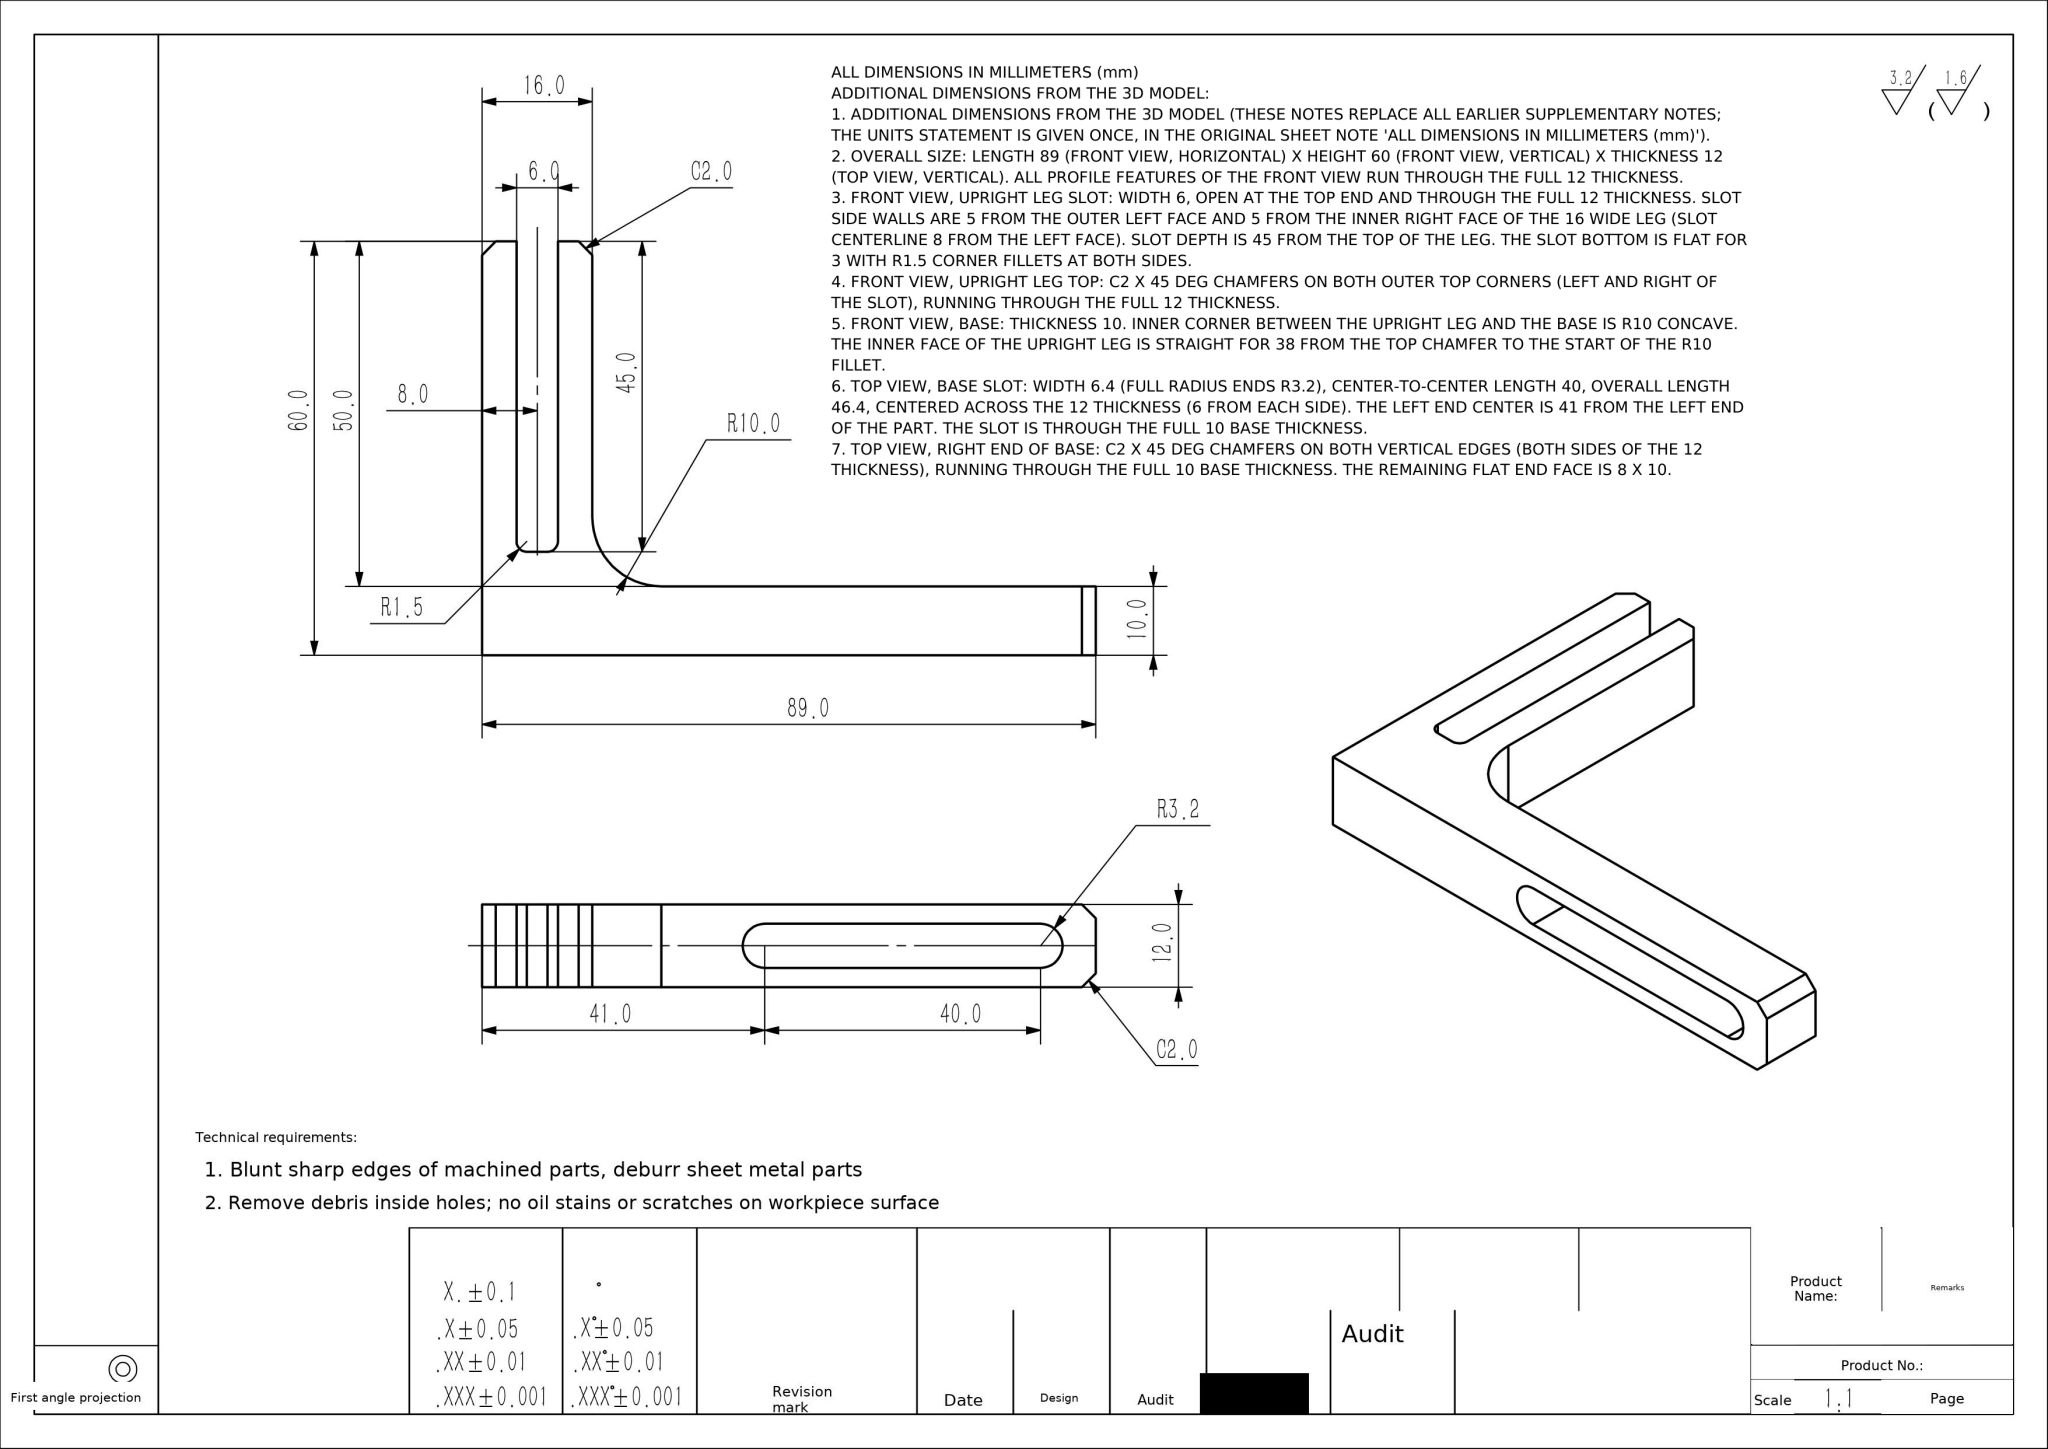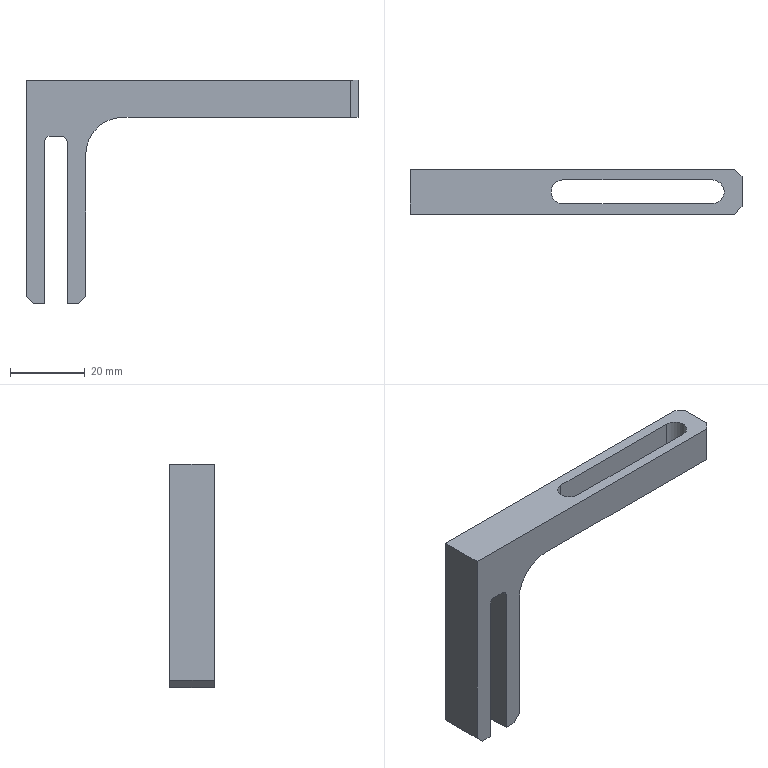Part | NX | mm | Right-Angle Slotted Post Bracket | 1 solid | 24 faces | box 89 x 12 x 60 mm | volume 14339 mm3 | plane 18 | cylinder 6 | commonest cylinder face diameters 6.4 x3 3 x2 20 x1
STEP:
#1=COLOUR_RGB('',1.,1.,1.);
#2=FILL_AREA_STYLE_COLOUR('',#1);
#3=FILL_AREA_STYLE('',(#2));
#4=SURFACE_STYLE_FILL_AREA(#3);
#5=SURFACE_SIDE_STYLE('',(#4));
#6=SURFACE_STYLE_USAGE(.BOTH.,#5);
#7=PRESENTATION_STYLE_ASSIGNMENT((#6));
#8=CARTESIAN_POINT('',(-6.7,6.,30.));
#9=VERTEX_POINT('',#8);
#10=CARTESIAN_POINT('',(-3.5,9.2,30.));
#11=VERTEX_POINT('',#10);
#12=CARTESIAN_POINT('',(-3.5,6.,30.));
#13=DIRECTION('',(-0.,0.,-1.));
#14=DIRECTION('',(-1.,0.,0.));
#15=AXIS2_PLACEMENT_3D('',#12,#13,#14);
#16=CIRCLE('',#15,3.2);
#17=EDGE_CURVE('',#9,#11,#16,.T.);
#18=ORIENTED_EDGE('',*,*,#17,.F.);
#19=CARTESIAN_POINT('',(-6.7,6.,20.));
#20=VERTEX_POINT('',#19);
#21=CARTESIAN_POINT('',(-6.7,6.,30.));
#22=DIRECTION('',(-0.,0.,-1.));
#23=VECTOR('',#22,1000.);
#24=LINE('',#21,#23);
#25=EDGE_CURVE('',#9,#20,#24,.T.);
#26=ORIENTED_EDGE('',*,*,#25,.T.);
#27=CARTESIAN_POINT('',(-3.5,9.2,20.));
#28=VERTEX_POINT('',#27);
#29=CARTESIAN_POINT('',(-3.5,6.,20.));
#30=DIRECTION('',(-0.,0.,-1.));
#31=DIRECTION('',(-1.,0.,0.));
#32=AXIS2_PLACEMENT_3D('',#29,#30,#31);
#33=CIRCLE('',#32,3.2);
#34=EDGE_CURVE('',#20,#28,#33,.T.);
#35=ORIENTED_EDGE('',*,*,#34,.T.);
#36=CARTESIAN_POINT('',(-3.5,9.2,30.));
#37=DIRECTION('',(-0.,0.,-1.));
#38=VECTOR('',#37,1000.);
#39=LINE('',#36,#38);
#40=EDGE_CURVE('',#11,#28,#39,.T.);
#41=ORIENTED_EDGE('',*,*,#40,.F.);
#42=EDGE_LOOP('',(#18,#26,#35,#41));
#43=FACE_OUTER_BOUND('',#42,.T.);
#44=CARTESIAN_POINT('',(-3.5,6.,30.));
#45=DIRECTION('',(-0.,0.,-1.));
#46=DIRECTION('',(-1.,0.,0.));
#47=AXIS2_PLACEMENT_3D('',#44,#45,#46);
#48=CYLINDRICAL_SURFACE('',#47,3.2);
#49=ADVANCED_FACE('',(#43),#48,.F.);
#50=CARTESIAN_POINT('',(-39.5,0.,-30.));
#51=VERTEX_POINT('',#50);
#52=CARTESIAN_POINT('',(-42.5,0.,-30.));
#53=VERTEX_POINT('',#52);
#54=CARTESIAN_POINT('',(-44.5,0.,-30.));
#55=DIRECTION('',(-1.,0.,0.));
#56=VECTOR('',#55,1000.);
#57=LINE('',#54,#56);
#58=EDGE_CURVE('',#51,#53,#57,.T.);
#59=ORIENTED_EDGE('',*,*,#58,.T.);
#60=CARTESIAN_POINT('',(-42.5,12.,-30.));
#61=VERTEX_POINT('',#60);
#62=CARTESIAN_POINT('',(-42.5,12.,-30.));
#63=DIRECTION('',(0.,1.,0.));
#64=VECTOR('',#63,1000.);
#65=LINE('',#62,#64);
#66=EDGE_CURVE('',#53,#61,#65,.T.);
#67=ORIENTED_EDGE('',*,*,#66,.T.);
#68=CARTESIAN_POINT('',(-39.5,12.,-30.));
#69=VERTEX_POINT('',#68);
#70=CARTESIAN_POINT('',(-44.5,12.,-30.));
#71=DIRECTION('',(-1.,0.,0.));
#72=VECTOR('',#71,1000.);
#73=LINE('',#70,#72);
#74=EDGE_CURVE('',#69,#61,#73,.T.);
#75=ORIENTED_EDGE('',*,*,#74,.F.);
#76=CARTESIAN_POINT('',(-39.5,0.,-30.));
#77=DIRECTION('',(0.,1.,0.));
#78=VECTOR('',#77,1000.);
#79=LINE('',#76,#78);
#80=EDGE_CURVE('',#51,#69,#79,.T.);
#81=ORIENTED_EDGE('',*,*,#80,.F.);
#82=EDGE_LOOP('',(#59,#67,#75,#81));
#83=FACE_OUTER_BOUND('',#82,.T.);
#84=CARTESIAN_POINT('',(-44.5,12.,-30.));
#85=DIRECTION('',(0.,0.,1.));
#86=DIRECTION('',(1.,0.,0.));
#87=AXIS2_PLACEMENT_3D('',#84,#85,#86);
#88=PLANE('',#87);
#89=ADVANCED_FACE('',(#83),#88,.F.);
#90=CARTESIAN_POINT('',(44.5,10.,30.));
#91=VERTEX_POINT('',#90);
#92=CARTESIAN_POINT('',(44.5,2.,30.));
#93=VERTEX_POINT('',#92);
#94=CARTESIAN_POINT('',(44.5,12.,30.));
#95=DIRECTION('',(0.,-1.,0.));
#96=VECTOR('',#95,1000.);
#97=LINE('',#94,#96);
#98=EDGE_CURVE('',#91,#93,#97,.T.);
#99=ORIENTED_EDGE('',*,*,#98,.T.);
#100=CARTESIAN_POINT('',(44.5,2.,20.));
#101=VERTEX_POINT('',#100);
#102=CARTESIAN_POINT('',(44.5,2.,20.));
#103=DIRECTION('',(0.,0.,-1.));
#104=VECTOR('',#103,1000.);
#105=LINE('',#102,#104);
#106=EDGE_CURVE('',#93,#101,#105,.T.);
#107=ORIENTED_EDGE('',*,*,#106,.T.);
#108=CARTESIAN_POINT('',(44.5,10.,20.));
#109=VERTEX_POINT('',#108);
#110=CARTESIAN_POINT('',(44.5,0.,20.));
#111=DIRECTION('',(0.,1.,0.));
#112=VECTOR('',#111,1000.);
#113=LINE('',#110,#112);
#114=EDGE_CURVE('',#101,#109,#113,.T.);
#115=ORIENTED_EDGE('',*,*,#114,.T.);
#116=CARTESIAN_POINT('',(44.5,10.,30.));
#117=DIRECTION('',(0.,0.,1.));
#118=VECTOR('',#117,1000.);
#119=LINE('',#116,#118);
#120=EDGE_CURVE('',#109,#91,#119,.T.);
#121=ORIENTED_EDGE('',*,*,#120,.T.);
#122=EDGE_LOOP('',(#99,#107,#115,#121));
#123=FACE_OUTER_BOUND('',#122,.T.);
#124=CARTESIAN_POINT('',(44.5,12.,30.));
#125=DIRECTION('',(-1.,0.,0.));
#126=DIRECTION('',(0.,0.,1.));
#127=AXIS2_PLACEMENT_3D('',#124,#125,#126);
#128=PLANE('',#127);
#129=ADVANCED_FACE('',(#123),#128,.F.);
#130=CARTESIAN_POINT('',(-30.5,12.,-30.));
#131=VERTEX_POINT('',#130);
#132=CARTESIAN_POINT('',(-33.5,12.,-30.));
#133=VERTEX_POINT('',#132);
#134=CARTESIAN_POINT('',(-44.5,12.,-30.));
#135=DIRECTION('',(-1.,0.,0.));
#136=VECTOR('',#135,1000.);
#137=LINE('',#134,#136);
#138=EDGE_CURVE('',#131,#133,#137,.T.);
#139=ORIENTED_EDGE('',*,*,#138,.F.);
#140=CARTESIAN_POINT('',(-30.5,0.,-30.));
#141=VERTEX_POINT('',#140);
#142=CARTESIAN_POINT('',(-30.5,12.,-30.));
#143=DIRECTION('',(0.,-1.,0.));
#144=VECTOR('',#143,1000.);
#145=LINE('',#142,#144);
#146=EDGE_CURVE('',#131,#141,#145,.T.);
#147=ORIENTED_EDGE('',*,*,#146,.T.);
#148=CARTESIAN_POINT('',(-33.5,0.,-30.));
#149=VERTEX_POINT('',#148);
#150=CARTESIAN_POINT('',(-44.5,0.,-30.));
#151=DIRECTION('',(-1.,0.,0.));
#152=VECTOR('',#151,1000.);
#153=LINE('',#150,#152);
#154=EDGE_CURVE('',#141,#149,#153,.T.);
#155=ORIENTED_EDGE('',*,*,#154,.T.);
#156=CARTESIAN_POINT('',(-33.5,0.,-30.));
#157=DIRECTION('',(0.,1.,0.));
#158=VECTOR('',#157,1000.);
#159=LINE('',#156,#158);
#160=EDGE_CURVE('',#149,#133,#159,.T.);
#161=ORIENTED_EDGE('',*,*,#160,.T.);
#162=EDGE_LOOP('',(#139,#147,#155,#161));
#163=FACE_OUTER_BOUND('',#162,.T.);
#164=CARTESIAN_POINT('',(-44.5,12.,-30.));
#165=DIRECTION('',(0.,0.,1.));
#166=DIRECTION('',(1.,0.,0.));
#167=AXIS2_PLACEMENT_3D('',#164,#165,#166);
#168=PLANE('',#167);
#169=ADVANCED_FACE('',(#163),#168,.F.);
#170=CARTESIAN_POINT('',(-44.5,12.,-28.));
#171=VERTEX_POINT('',#170);
#172=CARTESIAN_POINT('',(-44.5,12.,30.));
#173=VERTEX_POINT('',#172);
#174=CARTESIAN_POINT('',(-44.5,12.,30.));
#175=DIRECTION('',(0.,0.,1.));
#176=VECTOR('',#175,1000.);
#177=LINE('',#174,#176);
#178=EDGE_CURVE('',#171,#173,#177,.T.);
#179=ORIENTED_EDGE('',*,*,#178,.F.);
#180=CARTESIAN_POINT('',(-44.5,0.,-28.));
#181=VERTEX_POINT('',#180);
#182=CARTESIAN_POINT('',(-44.5,12.,-28.));
#183=DIRECTION('',(0.,-1.,0.));
#184=VECTOR('',#183,1000.);
#185=LINE('',#182,#184);
#186=EDGE_CURVE('',#171,#181,#185,.T.);
#187=ORIENTED_EDGE('',*,*,#186,.T.);
#188=CARTESIAN_POINT('',(-44.5,0.,30.));
#189=VERTEX_POINT('',#188);
#190=CARTESIAN_POINT('',(-44.5,0.,30.));
#191=DIRECTION('',(0.,0.,1.));
#192=VECTOR('',#191,1000.);
#193=LINE('',#190,#192);
#194=EDGE_CURVE('',#181,#189,#193,.T.);
#195=ORIENTED_EDGE('',*,*,#194,.T.);
#196=CARTESIAN_POINT('',(-44.5,12.,30.));
#197=DIRECTION('',(0.,-1.,0.));
#198=VECTOR('',#197,1000.);
#199=LINE('',#196,#198);
#200=EDGE_CURVE('',#173,#189,#199,.T.);
#201=ORIENTED_EDGE('',*,*,#200,.F.);
#202=EDGE_LOOP('',(#179,#187,#195,#201));
#203=FACE_OUTER_BOUND('',#202,.T.);
#204=CARTESIAN_POINT('',(-44.5,12.,30.));
#205=DIRECTION('',(1.,0.,0.));
#206=DIRECTION('',(0.,0.,-1.));
#207=AXIS2_PLACEMENT_3D('',#204,#205,#206);
#208=PLANE('',#207);
#209=ADVANCED_FACE('',(#203),#208,.F.);
#210=CARTESIAN_POINT('',(36.5,9.2,30.));
#211=VERTEX_POINT('',#210);
#212=CARTESIAN_POINT('',(36.5,9.2,30.));
#213=DIRECTION('',(1.,0.,0.));
#214=VECTOR('',#213,1000.);
#215=LINE('',#212,#214);
#216=EDGE_CURVE('',#11,#211,#215,.T.);
#217=ORIENTED_EDGE('',*,*,#216,.T.);
#218=CARTESIAN_POINT('',(36.5,2.8,30.));
#219=VERTEX_POINT('',#218);
#220=CARTESIAN_POINT('',(36.5,6.,30.));
#221=DIRECTION('',(-0.,0.,-1.));
#222=DIRECTION('',(-1.,0.,0.));
#223=AXIS2_PLACEMENT_3D('',#220,#221,#222);
#224=CIRCLE('',#223,3.2);
#225=EDGE_CURVE('',#211,#219,#224,.T.);
#226=ORIENTED_EDGE('',*,*,#225,.T.);
#227=CARTESIAN_POINT('',(-3.5,2.8,30.));
#228=VERTEX_POINT('',#227);
#229=CARTESIAN_POINT('',(36.5,2.8,30.));
#230=DIRECTION('',(-1.,0.,0.));
#231=VECTOR('',#230,1000.);
#232=LINE('',#229,#231);
#233=EDGE_CURVE('',#219,#228,#232,.T.);
#234=ORIENTED_EDGE('',*,*,#233,.T.);
#235=CARTESIAN_POINT('',(-3.5,6.,30.));
#236=DIRECTION('',(-0.,0.,-1.));
#237=DIRECTION('',(-1.,0.,0.));
#238=AXIS2_PLACEMENT_3D('',#235,#236,#237);
#239=CIRCLE('',#238,3.2);
#240=EDGE_CURVE('',#228,#9,#239,.T.);
#241=ORIENTED_EDGE('',*,*,#240,.T.);
#242=ORIENTED_EDGE('',*,*,#17,.T.);
#243=EDGE_LOOP('',(#217,#226,#234,#241,#242));
#244=FACE_BOUND('',#243,.T.);
#245=CARTESIAN_POINT('',(42.5,0.,30.));
#246=VERTEX_POINT('',#245);
#247=CARTESIAN_POINT('',(-44.5,0.,30.));
#248=DIRECTION('',(1.,0.,0.));
#249=VECTOR('',#248,1000.);
#250=LINE('',#247,#249);
#251=EDGE_CURVE('',#189,#246,#250,.T.);
#252=ORIENTED_EDGE('',*,*,#251,.T.);
#253=CARTESIAN_POINT('',(44.5,2.,30.));
#254=DIRECTION('',(0.7071,0.7071,0.));
#255=VECTOR('',#254,1000.);
#256=LINE('',#253,#255);
#257=EDGE_CURVE('',#246,#93,#256,.T.);
#258=ORIENTED_EDGE('',*,*,#257,.T.);
#259=ORIENTED_EDGE('',*,*,#98,.F.);
#260=CARTESIAN_POINT('',(42.5,12.,30.));
#261=VERTEX_POINT('',#260);
#262=CARTESIAN_POINT('',(42.5,12.,30.));
#263=DIRECTION('',(-0.7071,0.7071,0.));
#264=VECTOR('',#263,1000.);
#265=LINE('',#262,#264);
#266=EDGE_CURVE('',#91,#261,#265,.T.);
#267=ORIENTED_EDGE('',*,*,#266,.T.);
#268=CARTESIAN_POINT('',(-44.5,12.,30.));
#269=DIRECTION('',(1.,0.,0.));
#270=VECTOR('',#269,1000.);
#271=LINE('',#268,#270);
#272=EDGE_CURVE('',#173,#261,#271,.T.);
#273=ORIENTED_EDGE('',*,*,#272,.F.);
#274=ORIENTED_EDGE('',*,*,#200,.T.);
#275=EDGE_LOOP('',(#252,#258,#259,#267,#273,#274));
#276=FACE_OUTER_BOUND('',#275,.T.);
#277=CARTESIAN_POINT('',(-44.5,12.,30.));
#278=DIRECTION('',(0.,0.,-1.));
#279=DIRECTION('',(-1.,0.,0.));
#280=AXIS2_PLACEMENT_3D('',#277,#278,#279);
#281=PLANE('',#280);
#282=ADVANCED_FACE('',(#244,#276),#281,.F.);
#283=ORIENTED_EDGE('',*,*,#74,.T.);
#284=CARTESIAN_POINT('',(-44.5,12.,-28.));
#285=DIRECTION('',(-0.7071,0.,0.7071));
#286=VECTOR('',#285,1000.);
#287=LINE('',#284,#286);
#288=EDGE_CURVE('',#61,#171,#287,.T.);
#289=ORIENTED_EDGE('',*,*,#288,.T.);
#290=ORIENTED_EDGE('',*,*,#178,.T.);
#291=ORIENTED_EDGE('',*,*,#272,.T.);
#292=CARTESIAN_POINT('',(42.5,12.,20.));
#293=VERTEX_POINT('',#292);
#294=CARTESIAN_POINT('',(42.5,12.,0.));
#295=DIRECTION('',(0.,0.,-1.));
#296=VECTOR('',#295,1000.);
#297=LINE('',#294,#296);
#298=EDGE_CURVE('',#261,#293,#297,.T.);
#299=ORIENTED_EDGE('',*,*,#298,.T.);
#300=CARTESIAN_POINT('',(-18.5,12.,20.));
#301=VERTEX_POINT('',#300);
#302=CARTESIAN_POINT('',(44.5,12.,20.));
#303=DIRECTION('',(1.,0.,-0.));
#304=VECTOR('',#303,1000.);
#305=LINE('',#302,#304);
#306=EDGE_CURVE('',#301,#293,#305,.T.);
#307=ORIENTED_EDGE('',*,*,#306,.F.);
#308=CARTESIAN_POINT('',(-28.5,12.,10.));
#309=VERTEX_POINT('',#308);
#310=CARTESIAN_POINT('',(-18.5,12.,10.));
#311=DIRECTION('',(0.,-1.,0.));
#312=DIRECTION('',(0.,0.,-1.));
#313=AXIS2_PLACEMENT_3D('',#310,#311,#312);
#314=CIRCLE('',#313,10.);
#315=EDGE_CURVE('',#301,#309,#314,.T.);
#316=ORIENTED_EDGE('',*,*,#315,.T.);
#317=CARTESIAN_POINT('',(-28.5,12.,-28.));
#318=VERTEX_POINT('',#317);
#319=CARTESIAN_POINT('',(-28.5,12.,-30.));
#320=DIRECTION('',(0.,0.,1.));
#321=VECTOR('',#320,1000.);
#322=LINE('',#319,#321);
#323=EDGE_CURVE('',#318,#309,#322,.T.);
#324=ORIENTED_EDGE('',*,*,#323,.F.);
#325=CARTESIAN_POINT('',(-28.5,12.,-28.));
#326=DIRECTION('',(-0.7071,0.,-0.7071));
#327=VECTOR('',#326,1000.);
#328=LINE('',#325,#327);
#329=EDGE_CURVE('',#318,#131,#328,.T.);
#330=ORIENTED_EDGE('',*,*,#329,.T.);
#331=ORIENTED_EDGE('',*,*,#138,.T.);
#332=CARTESIAN_POINT('',(-33.5,12.,13.5));
#333=VERTEX_POINT('',#332);
#334=CARTESIAN_POINT('',(-33.5,12.,-30.));
#335=DIRECTION('',(0.,0.,-1.));
#336=VECTOR('',#335,1000.);
#337=LINE('',#334,#336);
#338=EDGE_CURVE('',#333,#133,#337,.T.);
#339=ORIENTED_EDGE('',*,*,#338,.F.);
#340=CARTESIAN_POINT('',(-35.,12.,15.));
#341=VERTEX_POINT('',#340);
#342=CARTESIAN_POINT('',(-35.,12.,13.5));
#343=DIRECTION('',(0.,-1.,0.));
#344=DIRECTION('',(0.,0.,-1.));
#345=AXIS2_PLACEMENT_3D('',#342,#343,#344);
#346=CIRCLE('',#345,1.5);
#347=EDGE_CURVE('',#333,#341,#346,.T.);
#348=ORIENTED_EDGE('',*,*,#347,.T.);
#349=CARTESIAN_POINT('',(-38.,12.,15.));
#350=VERTEX_POINT('',#349);
#351=CARTESIAN_POINT('',(-39.5,12.,15.));
#352=DIRECTION('',(1.,0.,0.));
#353=VECTOR('',#352,1000.);
#354=LINE('',#351,#353);
#355=EDGE_CURVE('',#350,#341,#354,.T.);
#356=ORIENTED_EDGE('',*,*,#355,.F.);
#357=CARTESIAN_POINT('',(-39.5,12.,13.5));
#358=VERTEX_POINT('',#357);
#359=CARTESIAN_POINT('',(-38.,12.,13.5));
#360=DIRECTION('',(0.,-1.,0.));
#361=DIRECTION('',(0.,0.,-1.));
#362=AXIS2_PLACEMENT_3D('',#359,#360,#361);
#363=CIRCLE('',#362,1.5);
#364=EDGE_CURVE('',#350,#358,#363,.T.);
#365=ORIENTED_EDGE('',*,*,#364,.T.);
#366=CARTESIAN_POINT('',(-39.5,12.,-30.));
#367=DIRECTION('',(0.,0.,1.));
#368=VECTOR('',#367,1000.);
#369=LINE('',#366,#368);
#370=EDGE_CURVE('',#69,#358,#369,.T.);
#371=ORIENTED_EDGE('',*,*,#370,.F.);
#372=EDGE_LOOP('',(#283,#289,#290,#291,#299,#307,#316,#324,#330,#331,#339,#348,#356,#365,#371));
#373=FACE_OUTER_BOUND('',#372,.T.);
#374=CARTESIAN_POINT('',(0.,12.,0.));
#375=DIRECTION('',(0.,-1.,0.));
#376=DIRECTION('',(0.,0.,-1.));
#377=AXIS2_PLACEMENT_3D('',#374,#375,#376);
#378=PLANE('',#377);
#379=ADVANCED_FACE('',(#373),#378,.F.);
#380=ORIENTED_EDGE('',*,*,#194,.F.);
#381=CARTESIAN_POINT('',(-36.25,0.,-36.25));
#382=DIRECTION('',(0.7071,0.,-0.7071));
#383=VECTOR('',#382,1000.);
#384=LINE('',#381,#383);
#385=EDGE_CURVE('',#181,#53,#384,.T.);
#386=ORIENTED_EDGE('',*,*,#385,.T.);
#387=ORIENTED_EDGE('',*,*,#58,.F.);
#388=CARTESIAN_POINT('',(-39.5,0.,13.5));
#389=VERTEX_POINT('',#388);
#390=CARTESIAN_POINT('',(-39.5,0.,-30.));
#391=DIRECTION('',(0.,0.,1.));
#392=VECTOR('',#391,1000.);
#393=LINE('',#390,#392);
#394=EDGE_CURVE('',#51,#389,#393,.T.);
#395=ORIENTED_EDGE('',*,*,#394,.T.);
#396=CARTESIAN_POINT('',(-38.,0.,15.));
#397=VERTEX_POINT('',#396);
#398=CARTESIAN_POINT('',(-38.,0.,13.5));
#399=DIRECTION('',(0.,1.,0.));
#400=DIRECTION('',(0.,0.,-1.));
#401=AXIS2_PLACEMENT_3D('',#398,#399,#400);
#402=CIRCLE('',#401,1.5);
#403=EDGE_CURVE('',#389,#397,#402,.T.);
#404=ORIENTED_EDGE('',*,*,#403,.T.);
#405=CARTESIAN_POINT('',(-35.,0.,15.));
#406=VERTEX_POINT('',#405);
#407=CARTESIAN_POINT('',(-39.5,0.,15.));
#408=DIRECTION('',(1.,0.,0.));
#409=VECTOR('',#408,1000.);
#410=LINE('',#407,#409);
#411=EDGE_CURVE('',#397,#406,#410,.T.);
#412=ORIENTED_EDGE('',*,*,#411,.T.);
#413=CARTESIAN_POINT('',(-33.5,0.,13.5));
#414=VERTEX_POINT('',#413);
#415=CARTESIAN_POINT('',(-35.,0.,13.5));
#416=DIRECTION('',(0.,1.,0.));
#417=DIRECTION('',(0.,0.,-1.));
#418=AXIS2_PLACEMENT_3D('',#415,#416,#417);
#419=CIRCLE('',#418,1.5);
#420=EDGE_CURVE('',#406,#414,#419,.T.);
#421=ORIENTED_EDGE('',*,*,#420,.T.);
#422=CARTESIAN_POINT('',(-33.5,0.,-30.));
#423=DIRECTION('',(0.,0.,-1.));
#424=VECTOR('',#423,1000.);
#425=LINE('',#422,#424);
#426=EDGE_CURVE('',#414,#149,#425,.T.);
#427=ORIENTED_EDGE('',*,*,#426,.T.);
#428=ORIENTED_EDGE('',*,*,#154,.F.);
#429=CARTESIAN_POINT('',(-28.5,0.,-28.));
#430=VERTEX_POINT('',#429);
#431=CARTESIAN_POINT('',(-0.25,0.,0.25));
#432=DIRECTION('',(0.7071,0.,0.7071));
#433=VECTOR('',#432,1000.);
#434=LINE('',#431,#433);
#435=EDGE_CURVE('',#141,#430,#434,.T.);
#436=ORIENTED_EDGE('',*,*,#435,.T.);
#437=CARTESIAN_POINT('',(-28.5,0.,10.));
#438=VERTEX_POINT('',#437);
#439=CARTESIAN_POINT('',(-28.5,0.,-30.));
#440=DIRECTION('',(0.,0.,1.));
#441=VECTOR('',#440,1000.);
#442=LINE('',#439,#441);
#443=EDGE_CURVE('',#430,#438,#442,.T.);
#444=ORIENTED_EDGE('',*,*,#443,.T.);
#445=CARTESIAN_POINT('',(-18.5,0.,20.));
#446=VERTEX_POINT('',#445);
#447=CARTESIAN_POINT('',(-18.5,0.,10.));
#448=DIRECTION('',(0.,1.,0.));
#449=DIRECTION('',(0.,0.,-1.));
#450=AXIS2_PLACEMENT_3D('',#447,#448,#449);
#451=CIRCLE('',#450,10.);
#452=EDGE_CURVE('',#438,#446,#451,.T.);
#453=ORIENTED_EDGE('',*,*,#452,.T.);
#454=CARTESIAN_POINT('',(42.5,0.,20.));
#455=VERTEX_POINT('',#454);
#456=CARTESIAN_POINT('',(44.5,0.,20.));
#457=DIRECTION('',(1.,0.,-0.));
#458=VECTOR('',#457,1000.);
#459=LINE('',#456,#458);
#460=EDGE_CURVE('',#446,#455,#459,.T.);
#461=ORIENTED_EDGE('',*,*,#460,.T.);
#462=CARTESIAN_POINT('',(42.5,0.,30.));
#463=DIRECTION('',(0.,0.,1.));
#464=VECTOR('',#463,1000.);
#465=LINE('',#462,#464);
#466=EDGE_CURVE('',#455,#246,#465,.T.);
#467=ORIENTED_EDGE('',*,*,#466,.T.);
#468=ORIENTED_EDGE('',*,*,#251,.F.);
#469=EDGE_LOOP('',(#380,#386,#387,#395,#404,#412,#421,#427,#428,#436,#444,#453,#461,#467,#468));
#470=FACE_OUTER_BOUND('',#469,.T.);
#471=CARTESIAN_POINT('',(0.,0.,0.));
#472=DIRECTION('',(0.,-1.,0.));
#473=DIRECTION('',(0.,0.,-1.));
#474=AXIS2_PLACEMENT_3D('',#471,#472,#473);
#475=PLANE('',#474);
#476=ADVANCED_FACE('',(#470),#475,.T.);
#477=CARTESIAN_POINT('',(36.5,2.8,20.));
#478=VERTEX_POINT('',#477);
#479=CARTESIAN_POINT('',(-3.5,2.8,20.));
#480=VERTEX_POINT('',#479);
#481=CARTESIAN_POINT('',(36.5,2.8,20.));
#482=DIRECTION('',(-1.,0.,0.));
#483=VECTOR('',#482,1000.);
#484=LINE('',#481,#483);
#485=EDGE_CURVE('',#478,#480,#484,.T.);
#486=ORIENTED_EDGE('',*,*,#485,.F.);
#487=CARTESIAN_POINT('',(36.5,9.2,20.));
#488=VERTEX_POINT('',#487);
#489=CARTESIAN_POINT('',(36.5,6.,20.));
#490=DIRECTION('',(-0.,0.,-1.));
#491=DIRECTION('',(-1.,0.,0.));
#492=AXIS2_PLACEMENT_3D('',#489,#490,#491);
#493=CIRCLE('',#492,3.2);
#494=EDGE_CURVE('',#488,#478,#493,.T.);
#495=ORIENTED_EDGE('',*,*,#494,.F.);
#496=CARTESIAN_POINT('',(36.5,9.2,20.));
#497=DIRECTION('',(1.,0.,0.));
#498=VECTOR('',#497,1000.);
#499=LINE('',#496,#498);
#500=EDGE_CURVE('',#28,#488,#499,.T.);
#501=ORIENTED_EDGE('',*,*,#500,.F.);
#502=ORIENTED_EDGE('',*,*,#34,.F.);
#503=CARTESIAN_POINT('',(-3.5,6.,20.));
#504=DIRECTION('',(-0.,0.,-1.));
#505=DIRECTION('',(-1.,0.,0.));
#506=AXIS2_PLACEMENT_3D('',#503,#504,#505);
#507=CIRCLE('',#506,3.2);
#508=EDGE_CURVE('',#480,#20,#507,.T.);
#509=ORIENTED_EDGE('',*,*,#508,.F.);
#510=EDGE_LOOP('',(#486,#495,#501,#502,#509));
#511=FACE_BOUND('',#510,.T.);
#512=ORIENTED_EDGE('',*,*,#114,.F.);
#513=CARTESIAN_POINT('',(44.5,2.,20.));
#514=DIRECTION('',(-0.7071,-0.7071,0.));
#515=VECTOR('',#514,1000.);
#516=LINE('',#513,#515);
#517=EDGE_CURVE('',#101,#455,#516,.T.);
#518=ORIENTED_EDGE('',*,*,#517,.T.);
#519=ORIENTED_EDGE('',*,*,#460,.F.);
#520=CARTESIAN_POINT('',(-18.5,12.,20.));
#521=DIRECTION('',(0.,1.,0.));
#522=VECTOR('',#521,1000.);
#523=LINE('',#520,#522);
#524=EDGE_CURVE('',#446,#301,#523,.T.);
#525=ORIENTED_EDGE('',*,*,#524,.T.);
#526=ORIENTED_EDGE('',*,*,#306,.T.);
#527=CARTESIAN_POINT('',(42.5,12.,20.));
#528=DIRECTION('',(0.7071,-0.7071,-0.));
#529=VECTOR('',#528,1000.);
#530=LINE('',#527,#529);
#531=EDGE_CURVE('',#293,#109,#530,.T.);
#532=ORIENTED_EDGE('',*,*,#531,.T.);
#533=EDGE_LOOP('',(#512,#518,#519,#525,#526,#532));
#534=FACE_OUTER_BOUND('',#533,.T.);
#535=CARTESIAN_POINT('',(44.5,0.,20.));
#536=DIRECTION('',(0.,0.,1.));
#537=DIRECTION('',(1.,0.,-0.));
#538=AXIS2_PLACEMENT_3D('',#535,#536,#537);
#539=PLANE('',#538);
#540=ADVANCED_FACE('',(#511,#534),#539,.F.);
#541=ORIENTED_EDGE('',*,*,#443,.F.);
#542=CARTESIAN_POINT('',(-28.5,0.,-28.));
#543=DIRECTION('',(0.,1.,0.));
#544=VECTOR('',#543,1000.);
#545=LINE('',#542,#544);
#546=EDGE_CURVE('',#430,#318,#545,.T.);
#547=ORIENTED_EDGE('',*,*,#546,.T.);
#548=ORIENTED_EDGE('',*,*,#323,.T.);
#549=CARTESIAN_POINT('',(-28.5,0.,10.));
#550=DIRECTION('',(0.,-1.,0.));
#551=VECTOR('',#550,1000.);
#552=LINE('',#549,#551);
#553=EDGE_CURVE('',#309,#438,#552,.T.);
#554=ORIENTED_EDGE('',*,*,#553,.T.);
#555=EDGE_LOOP('',(#541,#547,#548,#554));
#556=FACE_OUTER_BOUND('',#555,.T.);
#557=CARTESIAN_POINT('',(-28.5,0.,-30.));
#558=DIRECTION('',(-1.,0.,0.));
#559=DIRECTION('',(0.,0.,1.));
#560=AXIS2_PLACEMENT_3D('',#557,#558,#559);
#561=PLANE('',#560);
#562=ADVANCED_FACE('',(#556),#561,.F.);
#563=ORIENTED_EDGE('',*,*,#452,.F.);
#564=ORIENTED_EDGE('',*,*,#553,.F.);
#565=ORIENTED_EDGE('',*,*,#315,.F.);
#566=ORIENTED_EDGE('',*,*,#524,.F.);
#567=EDGE_LOOP('',(#563,#564,#565,#566));
#568=FACE_OUTER_BOUND('',#567,.T.);
#569=CARTESIAN_POINT('',(-18.5,0.,10.));
#570=DIRECTION('',(0.,-1.,0.));
#571=DIRECTION('',(0.,0.,-1.));
#572=AXIS2_PLACEMENT_3D('',#569,#570,#571);
#573=CYLINDRICAL_SURFACE('',#572,10.);
#574=ADVANCED_FACE('',(#568),#573,.F.);
#575=ORIENTED_EDGE('',*,*,#370,.T.);
#576=CARTESIAN_POINT('',(-39.5,0.,13.5));
#577=DIRECTION('',(0.,-1.,0.));
#578=VECTOR('',#577,1000.);
#579=LINE('',#576,#578);
#580=EDGE_CURVE('',#358,#389,#579,.T.);
#581=ORIENTED_EDGE('',*,*,#580,.T.);
#582=ORIENTED_EDGE('',*,*,#394,.F.);
#583=ORIENTED_EDGE('',*,*,#80,.T.);
#584=EDGE_LOOP('',(#575,#581,#582,#583));
#585=FACE_OUTER_BOUND('',#584,.T.);
#586=CARTESIAN_POINT('',(-39.5,0.,-30.));
#587=DIRECTION('',(-1.,0.,0.));
#588=DIRECTION('',(0.,0.,1.));
#589=AXIS2_PLACEMENT_3D('',#586,#587,#588);
#590=PLANE('',#589);
#591=ADVANCED_FACE('',(#585),#590,.F.);
#592=ORIENTED_EDGE('',*,*,#426,.F.);
#593=CARTESIAN_POINT('',(-33.5,12.,13.5));
#594=DIRECTION('',(0.,1.,0.));
#595=VECTOR('',#594,1000.);
#596=LINE('',#593,#595);
#597=EDGE_CURVE('',#414,#333,#596,.T.);
#598=ORIENTED_EDGE('',*,*,#597,.T.);
#599=ORIENTED_EDGE('',*,*,#338,.T.);
#600=ORIENTED_EDGE('',*,*,#160,.F.);
#601=EDGE_LOOP('',(#592,#598,#599,#600));
#602=FACE_OUTER_BOUND('',#601,.T.);
#603=CARTESIAN_POINT('',(-33.5,0.,-30.));
#604=DIRECTION('',(1.,0.,0.));
#605=DIRECTION('',(0.,0.,-1.));
#606=AXIS2_PLACEMENT_3D('',#603,#604,#605);
#607=PLANE('',#606);
#608=ADVANCED_FACE('',(#602),#607,.F.);
#609=ORIENTED_EDGE('',*,*,#411,.F.);
#610=CARTESIAN_POINT('',(-38.,12.,15.));
#611=DIRECTION('',(0.,1.,0.));
#612=VECTOR('',#611,1000.);
#613=LINE('',#610,#612);
#614=EDGE_CURVE('',#397,#350,#613,.T.);
#615=ORIENTED_EDGE('',*,*,#614,.T.);
#616=ORIENTED_EDGE('',*,*,#355,.T.);
#617=CARTESIAN_POINT('',(-35.,0.,15.));
#618=DIRECTION('',(0.,-1.,0.));
#619=VECTOR('',#618,1000.);
#620=LINE('',#617,#619);
#621=EDGE_CURVE('',#341,#406,#620,.T.);
#622=ORIENTED_EDGE('',*,*,#621,.T.);
#623=EDGE_LOOP('',(#609,#615,#616,#622));
#624=FACE_OUTER_BOUND('',#623,.T.);
#625=CARTESIAN_POINT('',(-39.5,0.,15.));
#626=DIRECTION('',(0.,0.,1.));
#627=DIRECTION('',(1.,0.,0.));
#628=AXIS2_PLACEMENT_3D('',#625,#626,#627);
#629=PLANE('',#628);
#630=ADVANCED_FACE('',(#624),#629,.F.);
#631=ORIENTED_EDGE('',*,*,#494,.T.);
#632=CARTESIAN_POINT('',(36.5,2.8,30.));
#633=DIRECTION('',(-0.,0.,-1.));
#634=VECTOR('',#633,1000.);
#635=LINE('',#632,#634);
#636=EDGE_CURVE('',#219,#478,#635,.T.);
#637=ORIENTED_EDGE('',*,*,#636,.F.);
#638=ORIENTED_EDGE('',*,*,#225,.F.);
#639=CARTESIAN_POINT('',(36.5,9.2,30.));
#640=DIRECTION('',(-0.,0.,-1.));
#641=VECTOR('',#640,1000.);
#642=LINE('',#639,#641);
#643=EDGE_CURVE('',#211,#488,#642,.T.);
#644=ORIENTED_EDGE('',*,*,#643,.T.);
#645=EDGE_LOOP('',(#631,#637,#638,#644));
#646=FACE_OUTER_BOUND('',#645,.T.);
#647=CARTESIAN_POINT('',(36.5,6.,30.));
#648=DIRECTION('',(-0.,0.,-1.));
#649=DIRECTION('',(-1.,0.,0.));
#650=AXIS2_PLACEMENT_3D('',#647,#648,#649);
#651=CYLINDRICAL_SURFACE('',#650,3.2);
#652=ADVANCED_FACE('',(#646),#651,.F.);
#653=ORIENTED_EDGE('',*,*,#500,.T.);
#654=ORIENTED_EDGE('',*,*,#643,.F.);
#655=ORIENTED_EDGE('',*,*,#216,.F.);
#656=ORIENTED_EDGE('',*,*,#40,.T.);
#657=EDGE_LOOP('',(#653,#654,#655,#656));
#658=FACE_OUTER_BOUND('',#657,.T.);
#659=CARTESIAN_POINT('',(36.5,9.2,30.));
#660=DIRECTION('',(-0.,1.,0.));
#661=DIRECTION('',(-1.,-0.,0.));
#662=AXIS2_PLACEMENT_3D('',#659,#660,#661);
#663=PLANE('',#662);
#664=ADVANCED_FACE('',(#658),#663,.F.);
#665=ORIENTED_EDGE('',*,*,#25,.F.);
#666=ORIENTED_EDGE('',*,*,#240,.F.);
#667=CARTESIAN_POINT('',(-3.5,2.8,30.));
#668=DIRECTION('',(-0.,0.,-1.));
#669=VECTOR('',#668,1000.);
#670=LINE('',#667,#669);
#671=EDGE_CURVE('',#228,#480,#670,.T.);
#672=ORIENTED_EDGE('',*,*,#671,.T.);
#673=ORIENTED_EDGE('',*,*,#508,.T.);
#674=EDGE_LOOP('',(#665,#666,#672,#673));
#675=FACE_OUTER_BOUND('',#674,.T.);
#676=CARTESIAN_POINT('',(-3.5,6.,30.));
#677=DIRECTION('',(-0.,0.,-1.));
#678=DIRECTION('',(-1.,0.,0.));
#679=AXIS2_PLACEMENT_3D('',#676,#677,#678);
#680=CYLINDRICAL_SURFACE('',#679,3.2);
#681=ADVANCED_FACE('',(#675),#680,.F.);
#682=ORIENTED_EDGE('',*,*,#485,.T.);
#683=ORIENTED_EDGE('',*,*,#671,.F.);
#684=ORIENTED_EDGE('',*,*,#233,.F.);
#685=ORIENTED_EDGE('',*,*,#636,.T.);
#686=EDGE_LOOP('',(#682,#683,#684,#685));
#687=FACE_OUTER_BOUND('',#686,.T.);
#688=CARTESIAN_POINT('',(36.5,2.8,30.));
#689=DIRECTION('',(-0.,-1.,0.));
#690=DIRECTION('',(1.,-0.,0.));
#691=AXIS2_PLACEMENT_3D('',#688,#689,#690);
#692=PLANE('',#691);
#693=ADVANCED_FACE('',(#687),#692,.F.);
#694=ORIENTED_EDGE('',*,*,#288,.F.);
#695=ORIENTED_EDGE('',*,*,#66,.F.);
#696=ORIENTED_EDGE('',*,*,#385,.F.);
#697=ORIENTED_EDGE('',*,*,#186,.F.);
#698=EDGE_LOOP('',(#694,#695,#696,#697));
#699=FACE_OUTER_BOUND('',#698,.T.);
#700=CARTESIAN_POINT('',(-44.5,12.,-28.));
#701=DIRECTION('',(0.7071,0.,0.7071));
#702=DIRECTION('',(0.,-1.,0.));
#703=AXIS2_PLACEMENT_3D('',#700,#701,#702);
#704=PLANE('',#703);
#705=ADVANCED_FACE('',(#699),#704,.F.);
#706=ORIENTED_EDGE('',*,*,#435,.F.);
#707=ORIENTED_EDGE('',*,*,#146,.F.);
#708=ORIENTED_EDGE('',*,*,#329,.F.);
#709=ORIENTED_EDGE('',*,*,#546,.F.);
#710=EDGE_LOOP('',(#706,#707,#708,#709));
#711=FACE_OUTER_BOUND('',#710,.T.);
#712=CARTESIAN_POINT('',(-28.5,0.,-28.));
#713=DIRECTION('',(-0.7071,0.,0.7071));
#714=DIRECTION('',(0.,1.,0.));
#715=AXIS2_PLACEMENT_3D('',#712,#713,#714);
#716=PLANE('',#715);
#717=ADVANCED_FACE('',(#711),#716,.F.);
#718=ORIENTED_EDGE('',*,*,#257,.F.);
#719=ORIENTED_EDGE('',*,*,#466,.F.);
#720=ORIENTED_EDGE('',*,*,#517,.F.);
#721=ORIENTED_EDGE('',*,*,#106,.F.);
#722=EDGE_LOOP('',(#718,#719,#720,#721));
#723=FACE_OUTER_BOUND('',#722,.T.);
#724=CARTESIAN_POINT('',(44.5,2.,30.));
#725=DIRECTION('',(0.7071,-0.7071,0.));
#726=DIRECTION('',(0.,0.,1.));
#727=AXIS2_PLACEMENT_3D('',#724,#725,#726);
#728=PLANE('',#727);
#729=ADVANCED_FACE('',(#723),#728,.T.);
#730=ORIENTED_EDGE('',*,*,#266,.F.);
#731=ORIENTED_EDGE('',*,*,#120,.F.);
#732=ORIENTED_EDGE('',*,*,#531,.F.);
#733=ORIENTED_EDGE('',*,*,#298,.F.);
#734=EDGE_LOOP('',(#730,#731,#732,#733));
#735=FACE_OUTER_BOUND('',#734,.T.);
#736=CARTESIAN_POINT('',(42.5,12.,0.));
#737=DIRECTION('',(-0.7071,-0.7071,0.));
#738=DIRECTION('',(0.,0.,-1.));
#739=AXIS2_PLACEMENT_3D('',#736,#737,#738);
#740=PLANE('',#739);
#741=ADVANCED_FACE('',(#735),#740,.F.);
#742=ORIENTED_EDGE('',*,*,#403,.F.);
#743=ORIENTED_EDGE('',*,*,#580,.F.);
#744=ORIENTED_EDGE('',*,*,#364,.F.);
#745=ORIENTED_EDGE('',*,*,#614,.F.);
#746=EDGE_LOOP('',(#742,#743,#744,#745));
#747=FACE_OUTER_BOUND('',#746,.T.);
#748=CARTESIAN_POINT('',(-38.,0.,13.5));
#749=DIRECTION('',(0.,-1.,0.));
#750=DIRECTION('',(0.,0.,-1.));
#751=AXIS2_PLACEMENT_3D('',#748,#749,#750);
#752=CYLINDRICAL_SURFACE('',#751,1.5);
#753=ADVANCED_FACE('',(#747),#752,.F.);
#754=ORIENTED_EDGE('',*,*,#420,.F.);
#755=ORIENTED_EDGE('',*,*,#621,.F.);
#756=ORIENTED_EDGE('',*,*,#347,.F.);
#757=ORIENTED_EDGE('',*,*,#597,.F.);
#758=EDGE_LOOP('',(#754,#755,#756,#757));
#759=FACE_OUTER_BOUND('',#758,.T.);
#760=CARTESIAN_POINT('',(-35.,0.,13.5));
#761=DIRECTION('',(0.,-1.,0.));
#762=DIRECTION('',(0.,0.,-1.));
#763=AXIS2_PLACEMENT_3D('',#760,#761,#762);
#764=CYLINDRICAL_SURFACE('',#763,1.5);
#765=ADVANCED_FACE('',(#759),#764,.F.);
#766=CLOSED_SHELL('',(#49,#89,#129,#169,#209,#282,#379,#476,#540,#562,#574,#591,#608,#630,#652,#664,#681,#693,#705,#717,#729,#741,#753,#765));
#767=MANIFOLD_SOLID_BREP('',#766);
#768=CARTESIAN_POINT('',(0.,0.,0.));
#769=DIRECTION('',(0.,0.,1.));
#770=DIRECTION('',(1.,0.,0.));
#771=AXIS2_PLACEMENT_3D('',#768,#769,#770);
#772=(LENGTH_UNIT()NAMED_UNIT(*)SI_UNIT(.MILLI.,.METRE.));
#773=UNCERTAINTY_MEASURE_WITH_UNIT(LENGTH_MEASURE(0.00001),#772,'','');
#774=(NAMED_UNIT(*)PLANE_ANGLE_UNIT()SI_UNIT($,.RADIAN.));
#775=(NAMED_UNIT(*)SI_UNIT($,.STERADIAN.)SOLID_ANGLE_UNIT());
#776=(GEOMETRIC_REPRESENTATION_CONTEXT(3)GLOBAL_UNCERTAINTY_ASSIGNED_CONTEXT((#773))GLOBAL_UNIT_ASSIGNED_CONTEXT((#772,#774,#775))REPRESENTATION_CONTEXT('',''));
#777=ADVANCED_BREP_SHAPE_REPRESENTATION('',(#767,#771),#776);
#778=STYLED_ITEM('',(#7),#777);
#779=PRESENTATION_LAYER_ASSIGNMENT('','',(#778));
#780=COLOUR_RGB('',1.,1.,1.);
#781=FILL_AREA_STYLE_COLOUR('',#780);
#782=FILL_AREA_STYLE('',(#781));
#783=SURFACE_STYLE_FILL_AREA(#782);
#784=SURFACE_SIDE_STYLE('',(#783));
#785=SURFACE_STYLE_USAGE(.BOTH.,#784);
#786=PRESENTATION_STYLE_ASSIGNMENT((#785));
#787=STYLED_ITEM('',(#786),#767);
#788=(LENGTH_UNIT()NAMED_UNIT(*)SI_UNIT(.MILLI.,.METRE.));
#789=UNCERTAINTY_MEASURE_WITH_UNIT(LENGTH_MEASURE(0.00001),#788,'','');
#790=(NAMED_UNIT(*)PLANE_ANGLE_UNIT()SI_UNIT($,.RADIAN.));
#791=(NAMED_UNIT(*)SI_UNIT($,.STERADIAN.)SOLID_ANGLE_UNIT());
#792=(GEOMETRIC_REPRESENTATION_CONTEXT(3)GLOBAL_UNCERTAINTY_ASSIGNED_CONTEXT((#789))GLOBAL_UNIT_ASSIGNED_CONTEXT((#788,#790,#791))REPRESENTATION_CONTEXT('',''));
#793=MECHANICAL_DESIGN_GEOMETRIC_PRESENTATION_REPRESENTATION('',(#787),#792);
#794=(LENGTH_UNIT()NAMED_UNIT(*)SI_UNIT(.MILLI.,.METRE.));
#795=UNCERTAINTY_MEASURE_WITH_UNIT(LENGTH_MEASURE(0.00001),#794,'','');
#796=(NAMED_UNIT(*)PLANE_ANGLE_UNIT()SI_UNIT($,.RADIAN.));
#797=(NAMED_UNIT(*)SI_UNIT($,.STERADIAN.)SOLID_ANGLE_UNIT());
#798=(GEOMETRIC_REPRESENTATION_CONTEXT(3)GLOBAL_UNCERTAINTY_ASSIGNED_CONTEXT((#795))GLOBAL_UNIT_ASSIGNED_CONTEXT((#794,#796,#797))REPRESENTATION_CONTEXT('',''));
#799=MECHANICAL_DESIGN_GEOMETRIC_PRESENTATION_REPRESENTATION('',(#778),#798);
#800=PRESENTATION_LAYER_ASSIGNMENT('','',(#787));